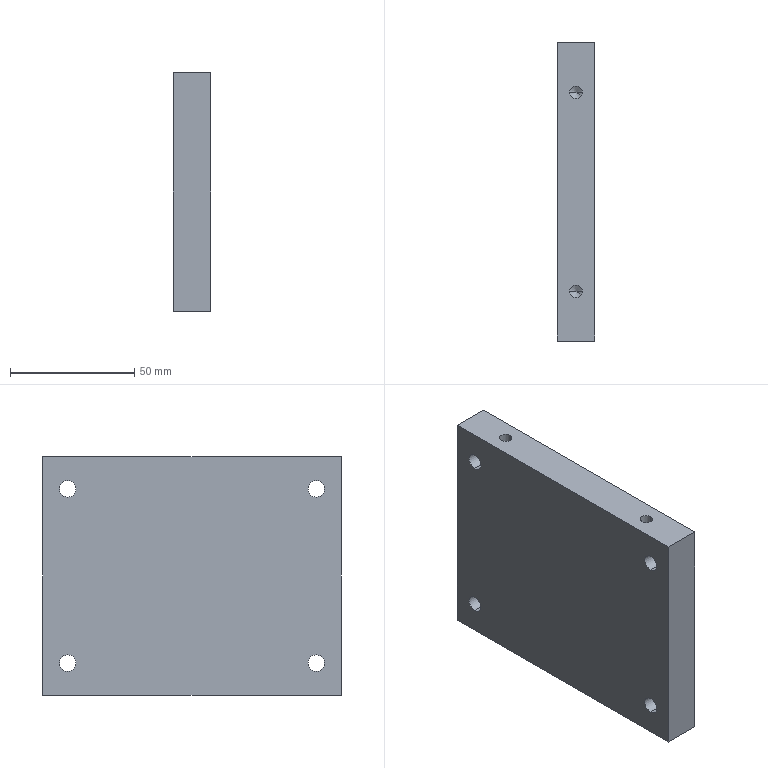Component | SolidWorks | WT-FLD-EJG-1212-00-007-1 | 1 solid | 42 faces | box 15 x 120 x 96 mm | volume 167973 mm3 | cylinder 24 | plane 10 | cone 8 | commonest cylinder face diameters 11 x8 6.6 x8 5 x8 | material AISI 1045 Steel, cold drawn
build123d program:
from build123d import *

# Parameters (mm, degrees)
SKETCH1_W                                       = 96
SKETCH1_H                                       = 120
BOSS_EXTRUDE1_DEPTH                             = 15
M6_TAPPED_HOLE1_AT_2_COUNT                      = 2
M6_TAPPED_HOLE1_AT_2_PITCH                      = 80
M6_HEX_SOCKET_HEAD_CAP_SCREW_CBORE1_D           = 6.6
M6_HEX_SOCKET_HEAD_CAP_SCREW_CBORE1_CBORE_D     = 11
M6_HEX_SOCKET_HEAD_CAP_SCREW_CBORE1_CBORE_DEPTH = 6.4


with BuildPart() as part:
    # Sketch1 → Boss-Extrude1 (new body)
    with BuildSketch(Plane.XY):
        Rectangle(SKETCH1_W, SKETCH1_H)
    extrude(amount=BOSS_EXTRUDE1_DEPTH)

    # Sketch2 → M6 Tapped Hole1 (revolve, cut)
    with BuildSketch(Plane(origin=(48, 40, 7.5), x_dir=(0, 0, -1), z_dir=(0, 1, 0))):
        Polygon((0, 0), (0, 16.502), (2.5, 15), (2.5, 0), align=None)
    m6_tapped_hole1 = revolve(axis=Axis((54.35, 40, 7.5), (-1, 0, 0)), mode=Mode.SUBTRACT)

    # M6 Tapped Hole1 at 2: M6 Tapped Hole1 ×2
    with Locations(*[(0, -i * M6_TAPPED_HOLE1_AT_2_PITCH, 0) for i in range(1, M6_TAPPED_HOLE1_AT_2_COUNT)]):
        add(m6_tapped_hole1, mode=Mode.SUBTRACT)

    # Mirror1: M6 Tapped Hole1 across plane
    add(m6_tapped_hole1.mirror(Plane(origin=(0, 0, 0), x_dir=(0, 0, 1), z_dir=(1, 0, 0))), mode=Mode.SUBTRACT)

    # Mirror1 copy 1 sketch → Mirror1 copy 1 (revolve, cut)
    with BuildSketch(Plane(origin=(-48, -40, 7.5), x_dir=(0, 0, -1), z_dir=(0, 1, 0))):
        Polygon((0, 0), (0, -16.502), (2.5, -15), (2.5, 0), align=None)
    revolve(axis=Axis((-54.35, -40, 7.5), (-1, 0, 0)), mode=Mode.SUBTRACT)

    # M6 Hex Socket Head Cap Screw CBORE1 (through all)
    with Locations(Plane.XY.offset(15)):
        with Locations((-35, 50), (-35, -50), (35, 50), (35, -50)):
            CounterBoreHole(M6_HEX_SOCKET_HEAD_CAP_SCREW_CBORE1_D / 2, M6_HEX_SOCKET_HEAD_CAP_SCREW_CBORE1_CBORE_D / 2, M6_HEX_SOCKET_HEAD_CAP_SCREW_CBORE1_CBORE_DEPTH)


solid = part.part

# Placed as in the assembly
solid = solid.moved(Location((-127, 0, 0), (0, 90, 0)))